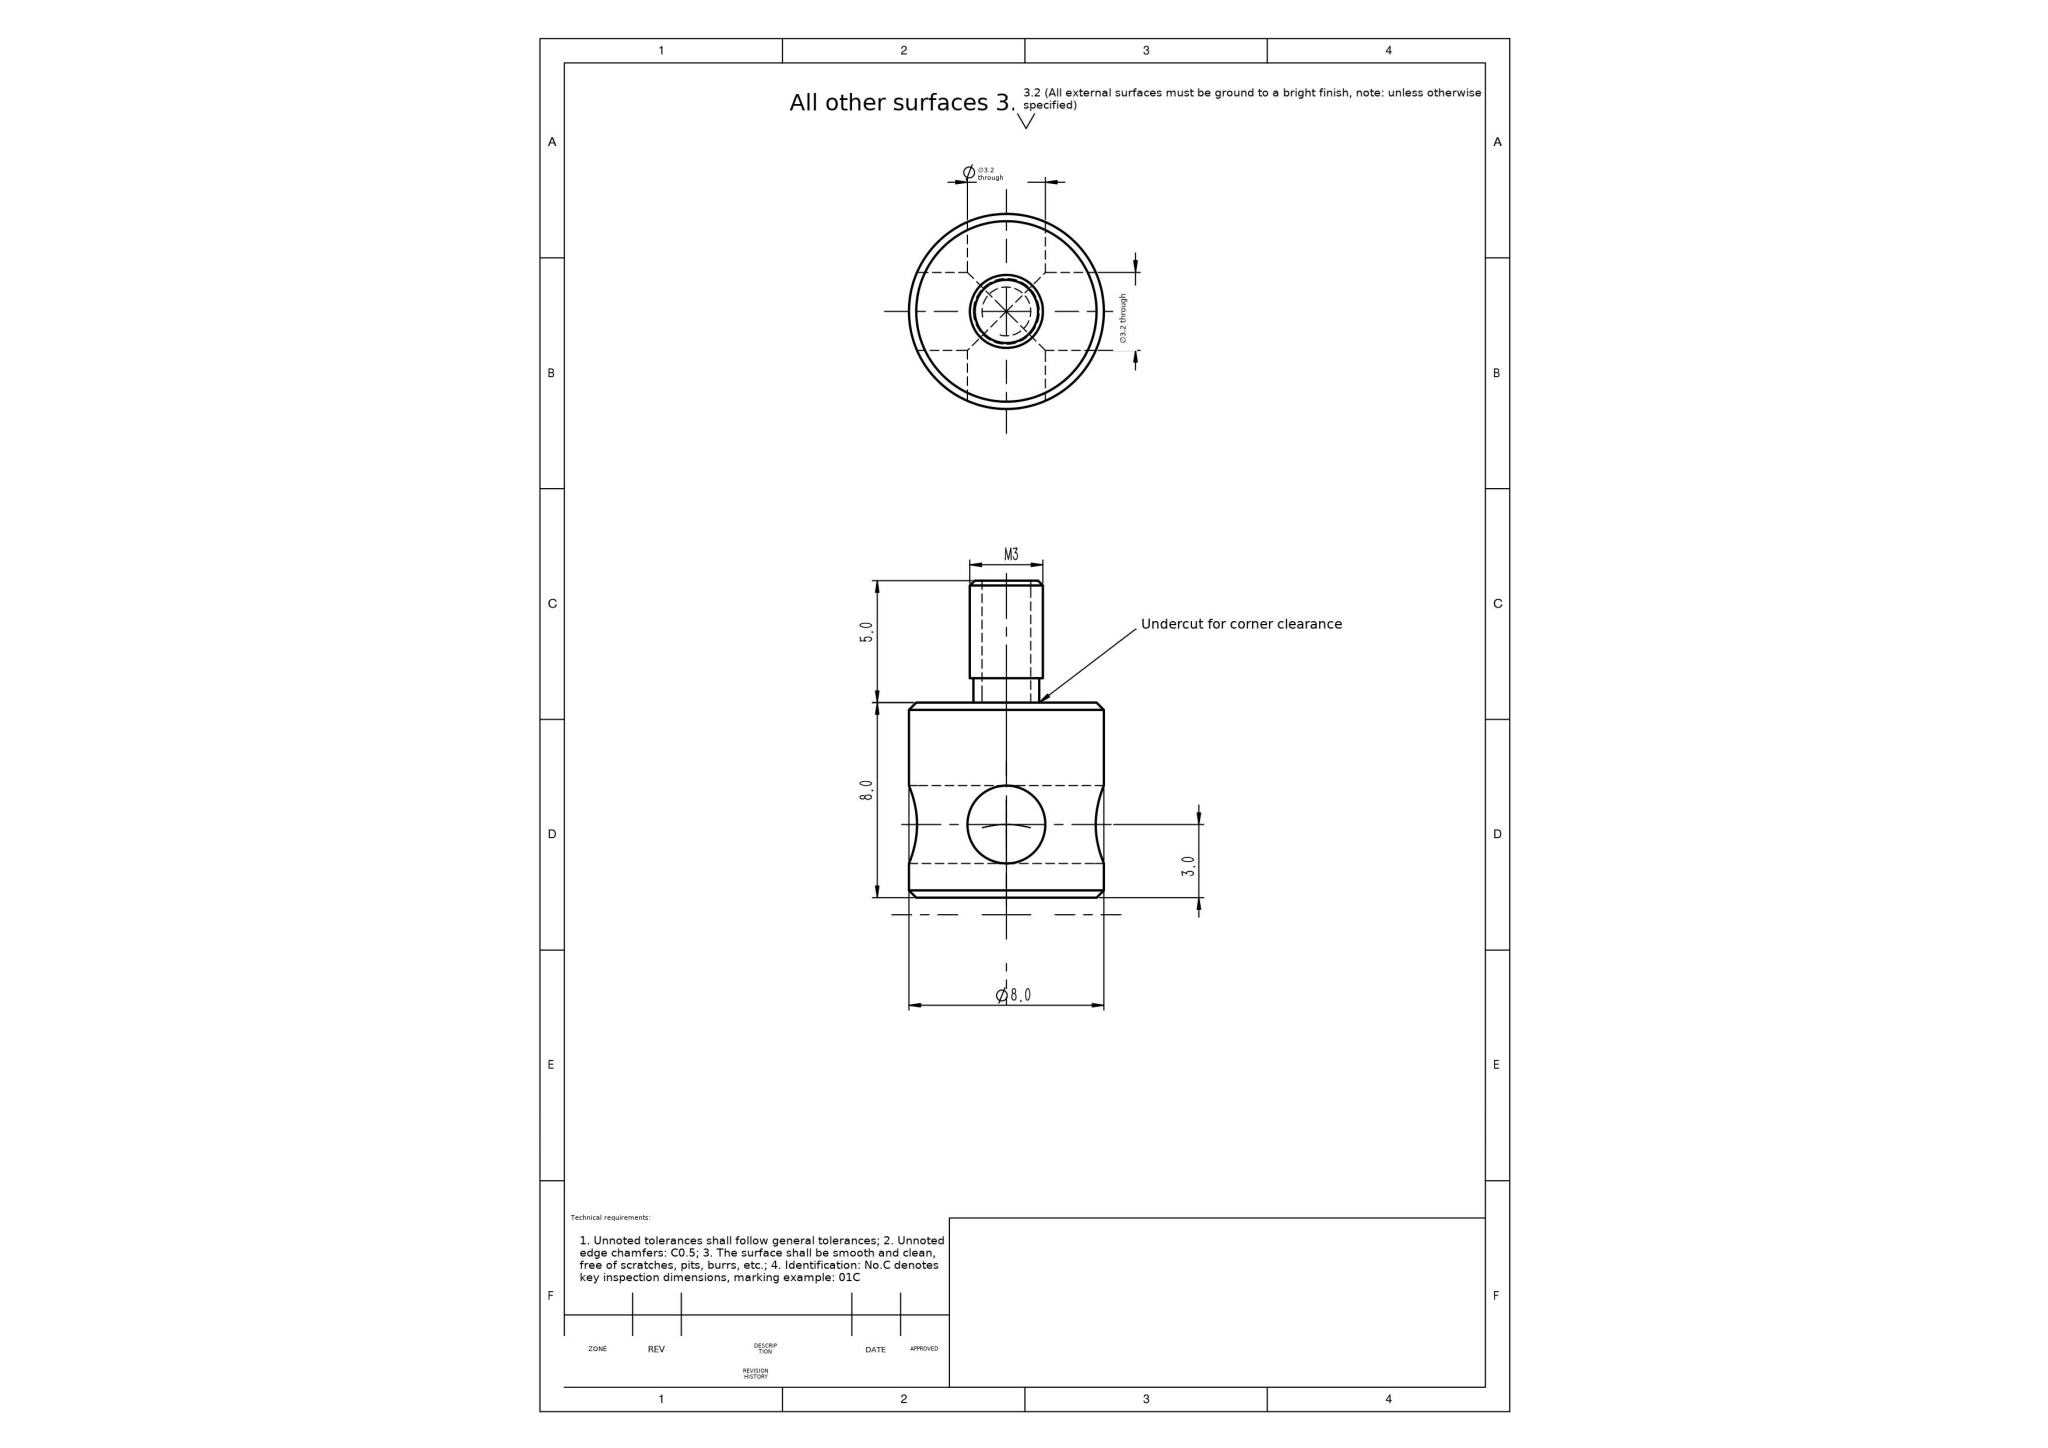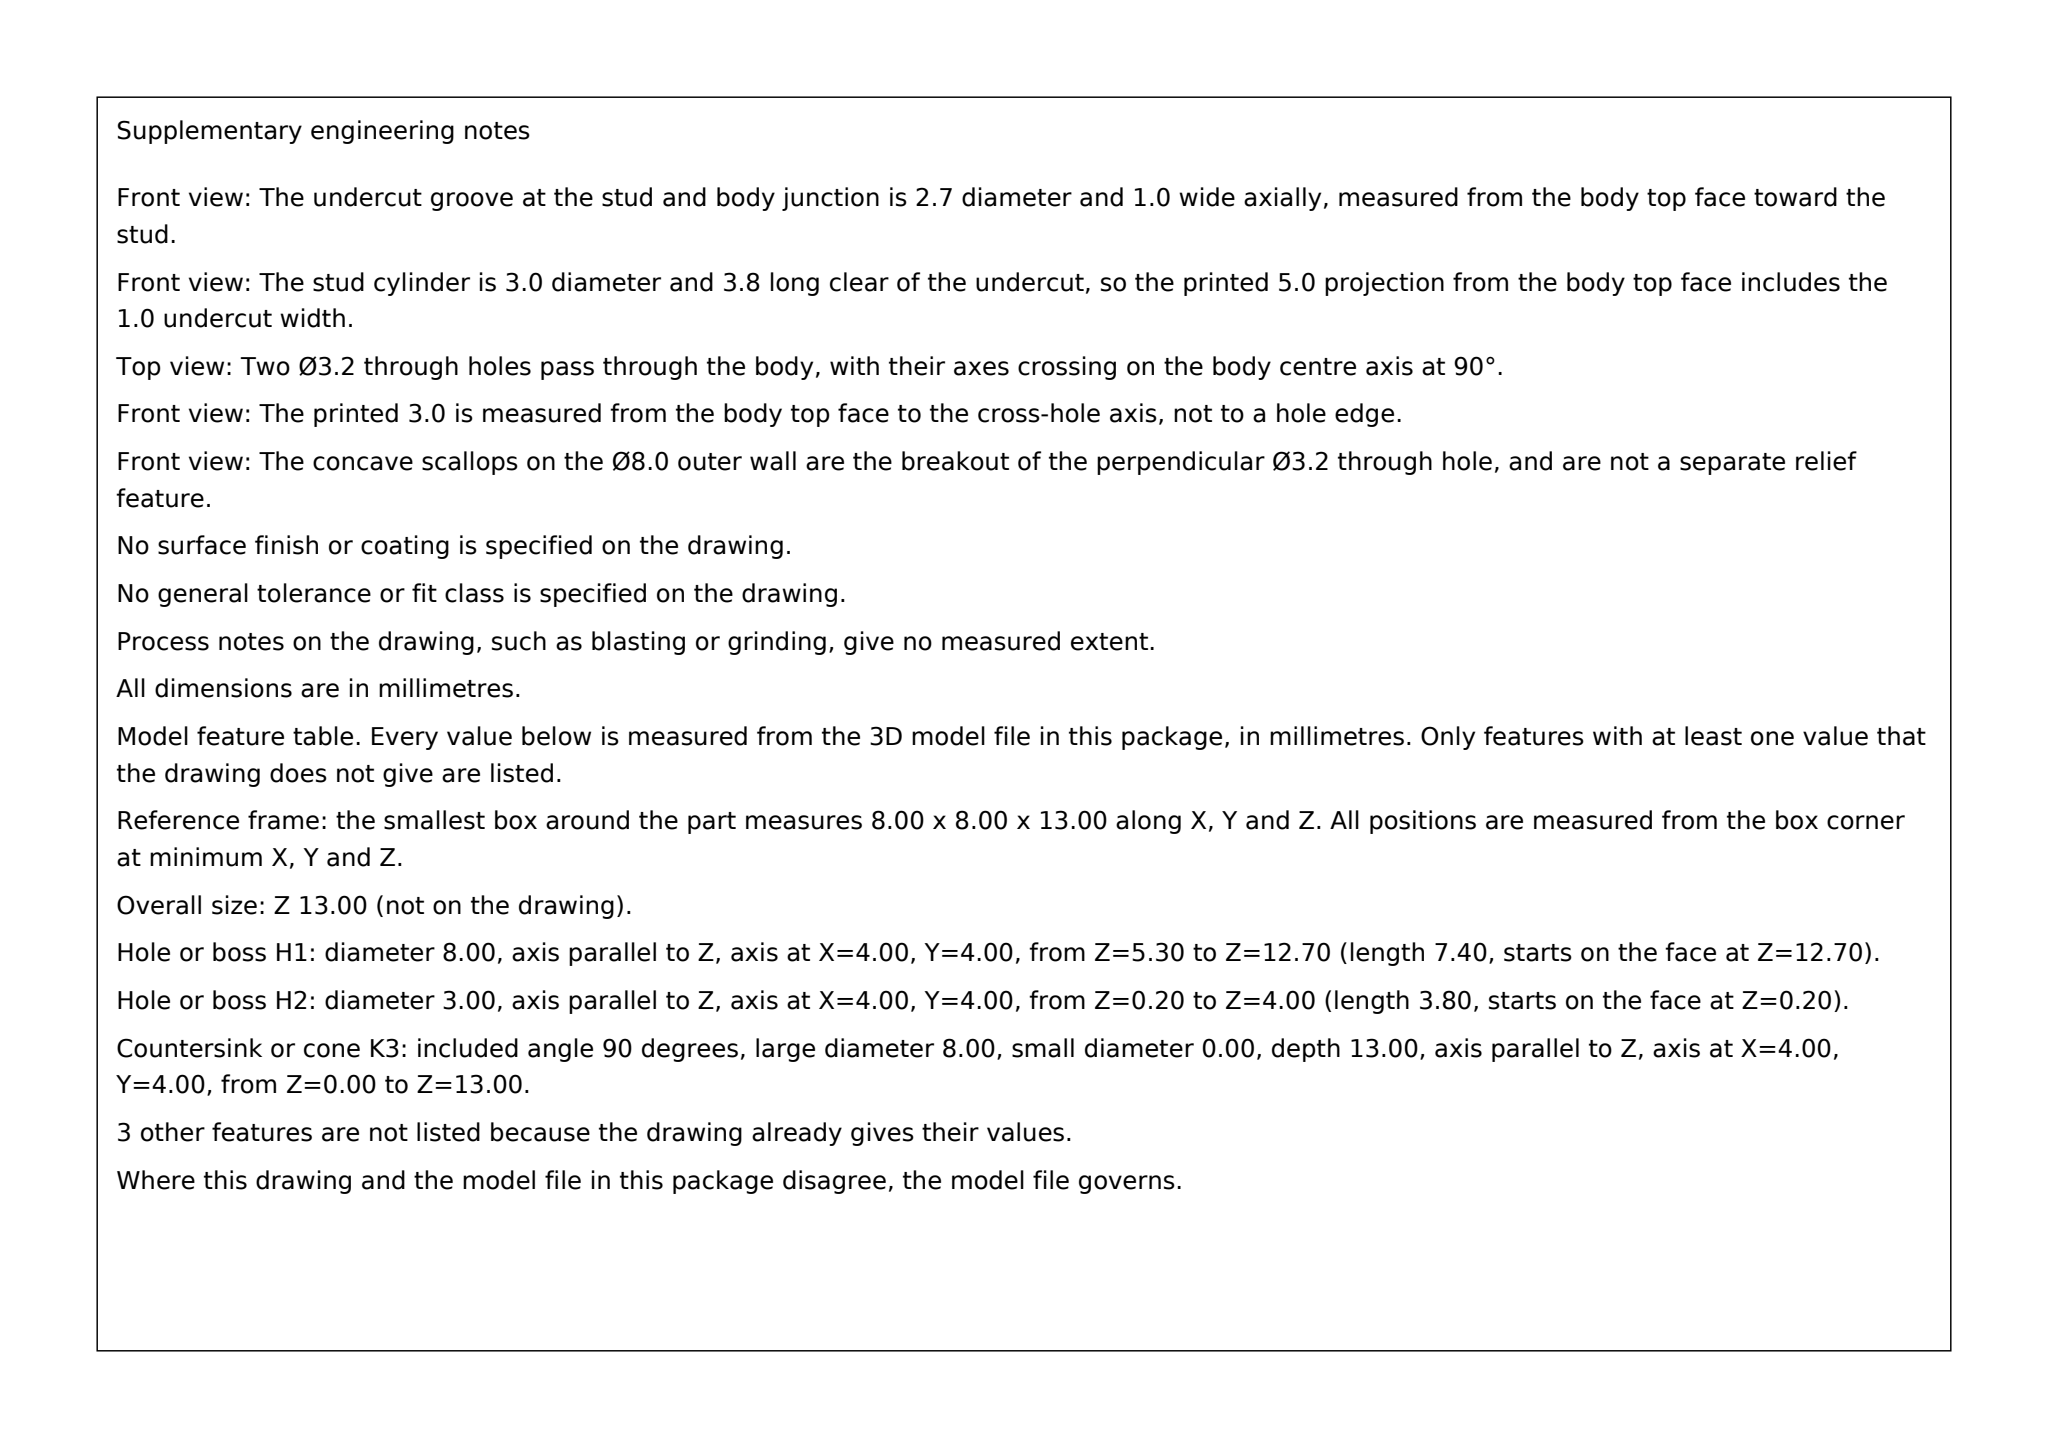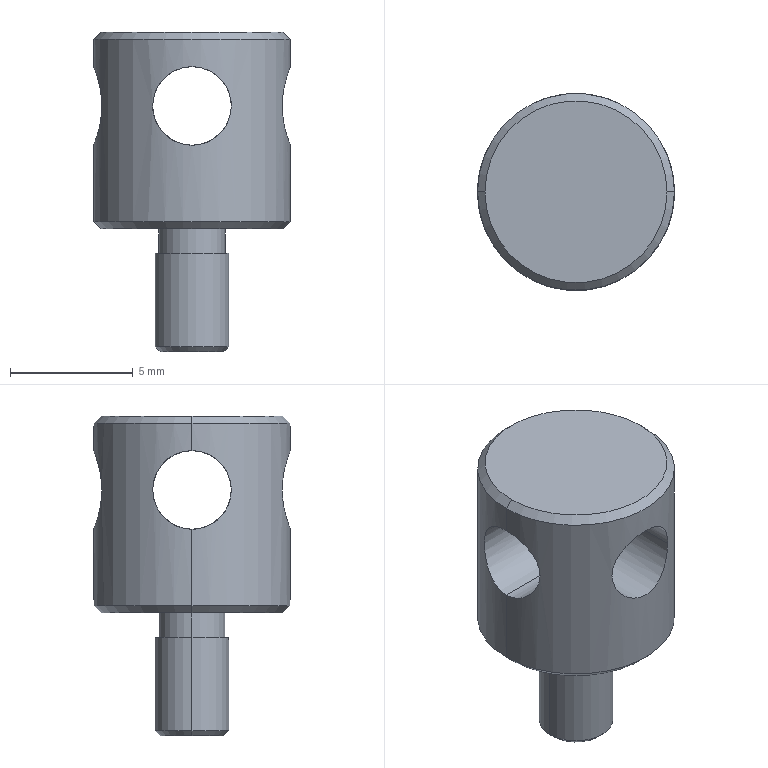Part | SolidWorks | mm | 1 solid | 24 faces | box 8 x 8 x 13 mm | volume 330 mm3 | cylinder 14 | cone 6 | plane 4 | commonest cylinder face diameters 3.2 x8 3 x2 2.7 x2 8 x2
build123d program:
from build123d import *

# Parameters (mm, degrees)
SKETCH1_R           = 1.5
BOSS_EXTRUDE1_DEPTH = 5
SKETCH2_R           = 4
BOSS_EXTRUDE2_DEPTH = 8
SKETCH3_R           = 1.6
CUT_EXTRUDE1_DEPTH  = 15.177
CUT_EXTRUDE2_START  = 1
SKETCH4_R           = 4
SKETCH4_R_2         = 1.35
CUT_EXTRUDE2_DEPTH  = 1
CIRPATTERN1_COUNT   = 2
CIRPATTERN1_ANGLE   = 90
CHAMFER1_SIZE       = 0.3
CHAMFER2_SIZE       = 0.2


with BuildPart() as part:
    # Sketch1 → Boss-Extrude1 (new body)
    with BuildSketch(Plane.XY):
        Circle(SKETCH1_R)
    extrude(amount=BOSS_EXTRUDE1_DEPTH)

    # Sketch2 → Boss-Extrude2 (add)
    with BuildSketch(Plane.XY.offset(5)):
        Circle(SKETCH2_R)
    extrude(amount=BOSS_EXTRUDE2_DEPTH)

    # Sketch3 → Cut-Extrude1 (cut, symmetric)
    with BuildSketch(Plane(origin=(0, 0, 0), x_dir=(0, 0, -1), z_dir=(1, 0, 0))):
        with Locations((-10, 0)):
            Circle(SKETCH3_R)
    cut_extrude1 = extrude(amount=CUT_EXTRUDE1_DEPTH, both=True, mode=Mode.SUBTRACT)

    # Sketch4 → Cut-Extrude2 (cut)
    with BuildSketch(Plane(origin=(0, 0, 5), x_dir=(-1, 0, 0), z_dir=(0, 0, -1)).offset(CUT_EXTRUDE2_START)):
        with Locations(Location((0, 0, 0), (0, 0, 180))):
            Circle(SKETCH4_R)
        Circle(SKETCH4_R_2, mode=Mode.SUBTRACT)
    extrude(amount=-CUT_EXTRUDE2_DEPTH, mode=Mode.SUBTRACT)

    # CirPattern1: Cut-Extrude1 ×2 about axis
    cirpattern1_axis = Axis((0, 0, 13), (0, 0, -1))
    for i in range(1, CIRPATTERN1_COUNT):
        add(cut_extrude1.rotate(cirpattern1_axis, i * CIRPATTERN1_ANGLE / (CIRPATTERN1_COUNT - 1)), mode=Mode.SUBTRACT)

    # Chamfer1
    chamfer1_edges = [part.edges().sort_by_distance(p)[0] for p in [
        (-4, 0, 5),
        (-4, 0, 13),
    ]]
    chamfer(chamfer1_edges, length=CHAMFER1_SIZE)

    # Chamfer2
    chamfer2_edges = [part.edges().sort_by_distance(p)[0] for p in [
        (-1.5, 0, 0),
    ]]
    chamfer(chamfer2_edges, length=CHAMFER2_SIZE)


solid = part.part